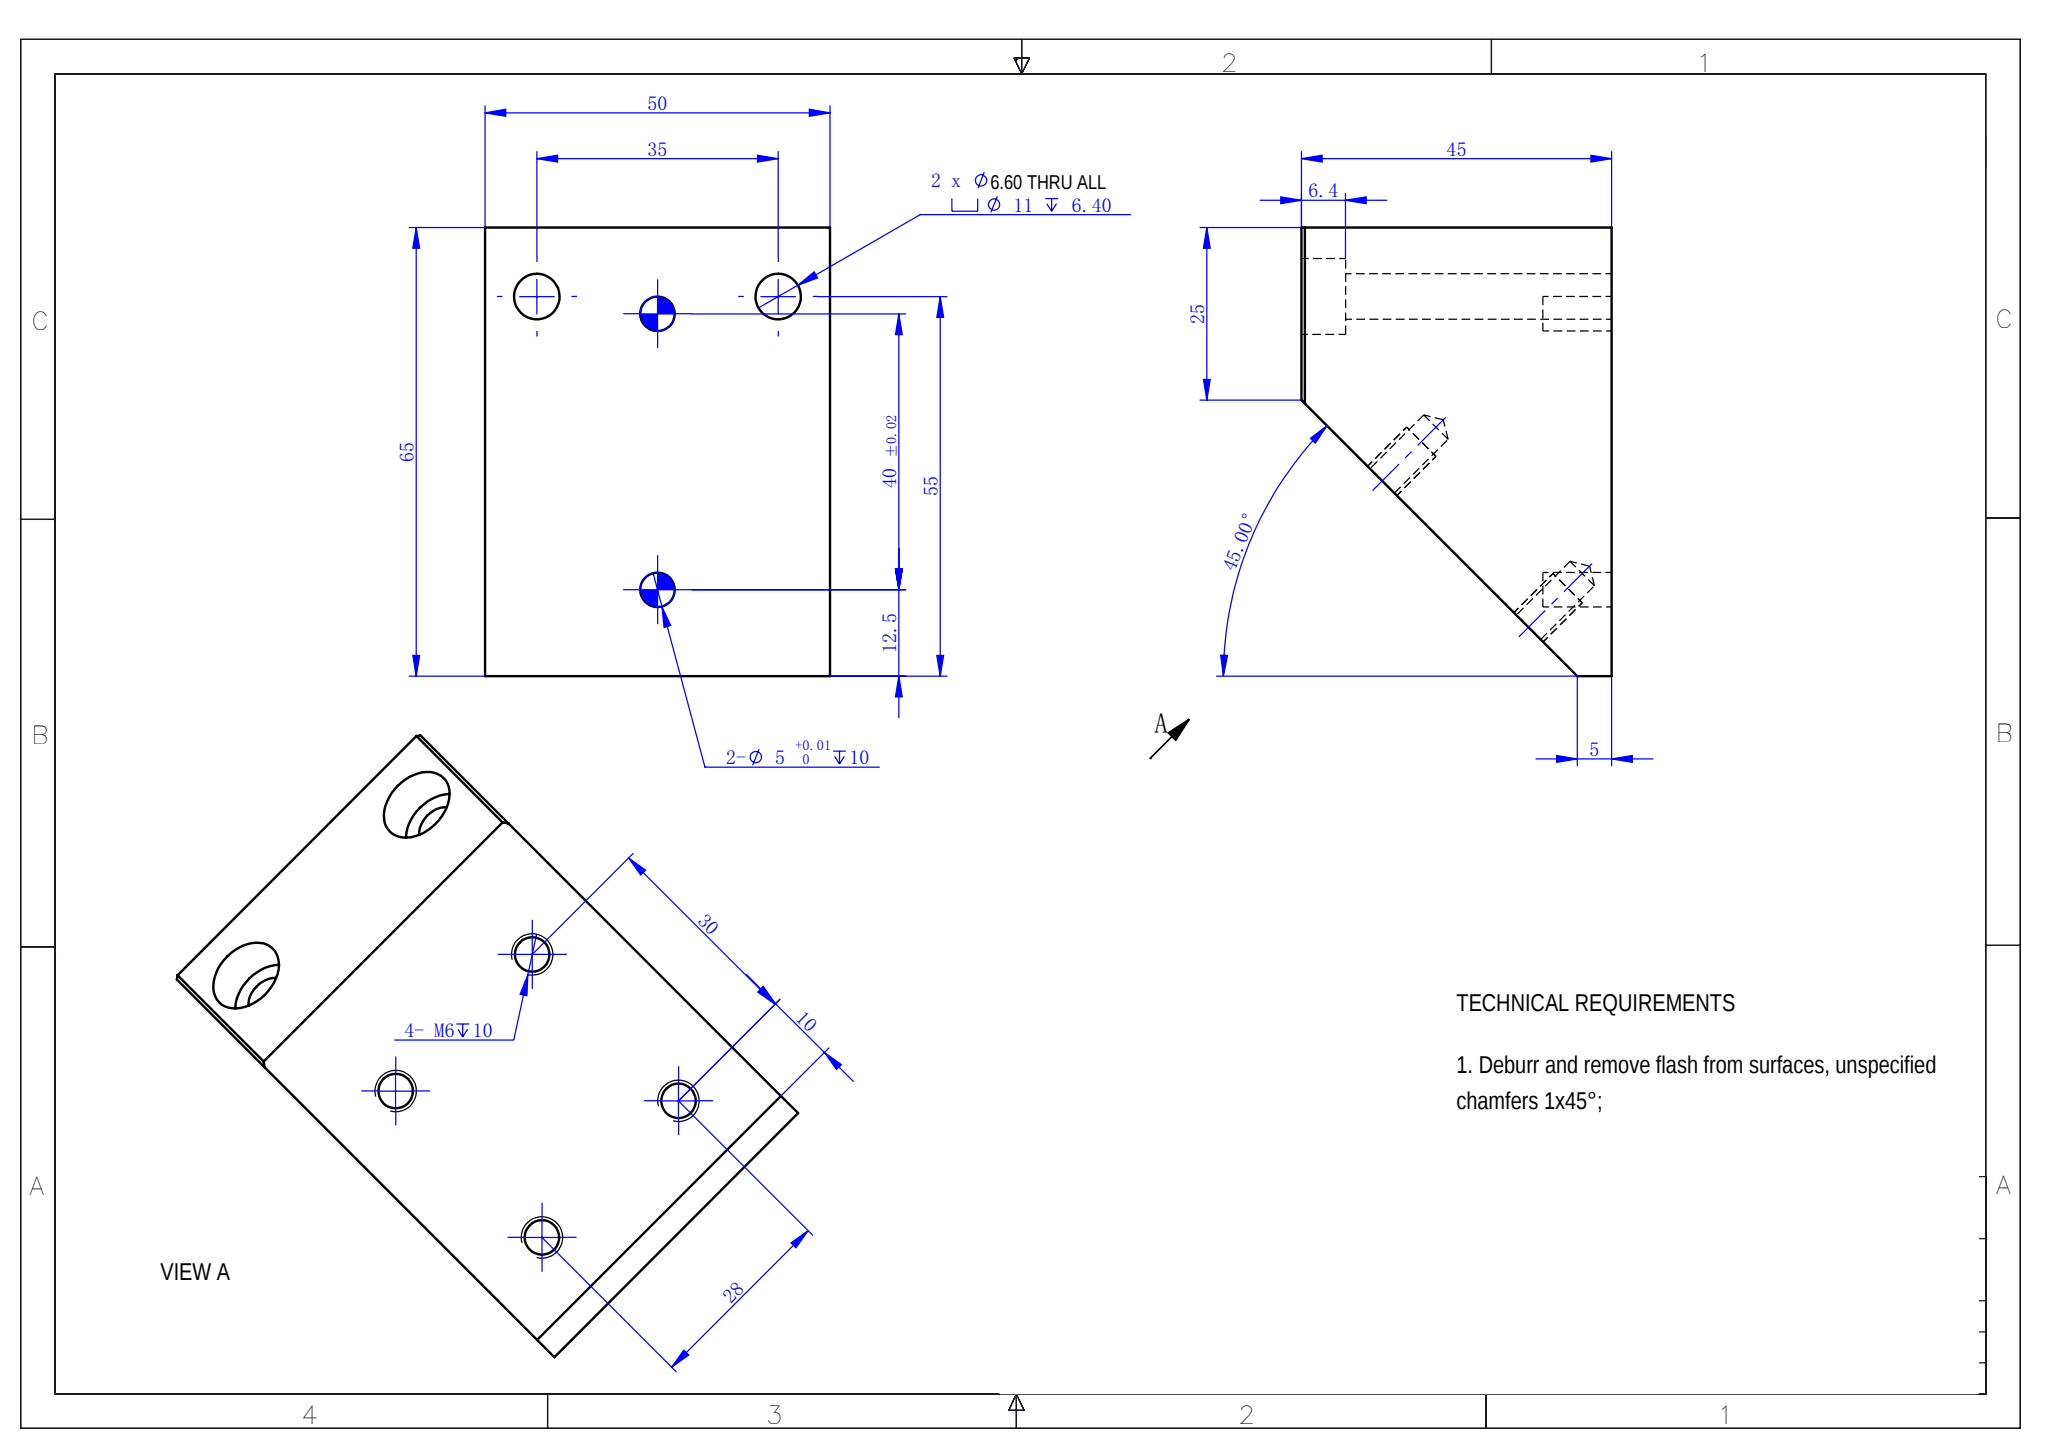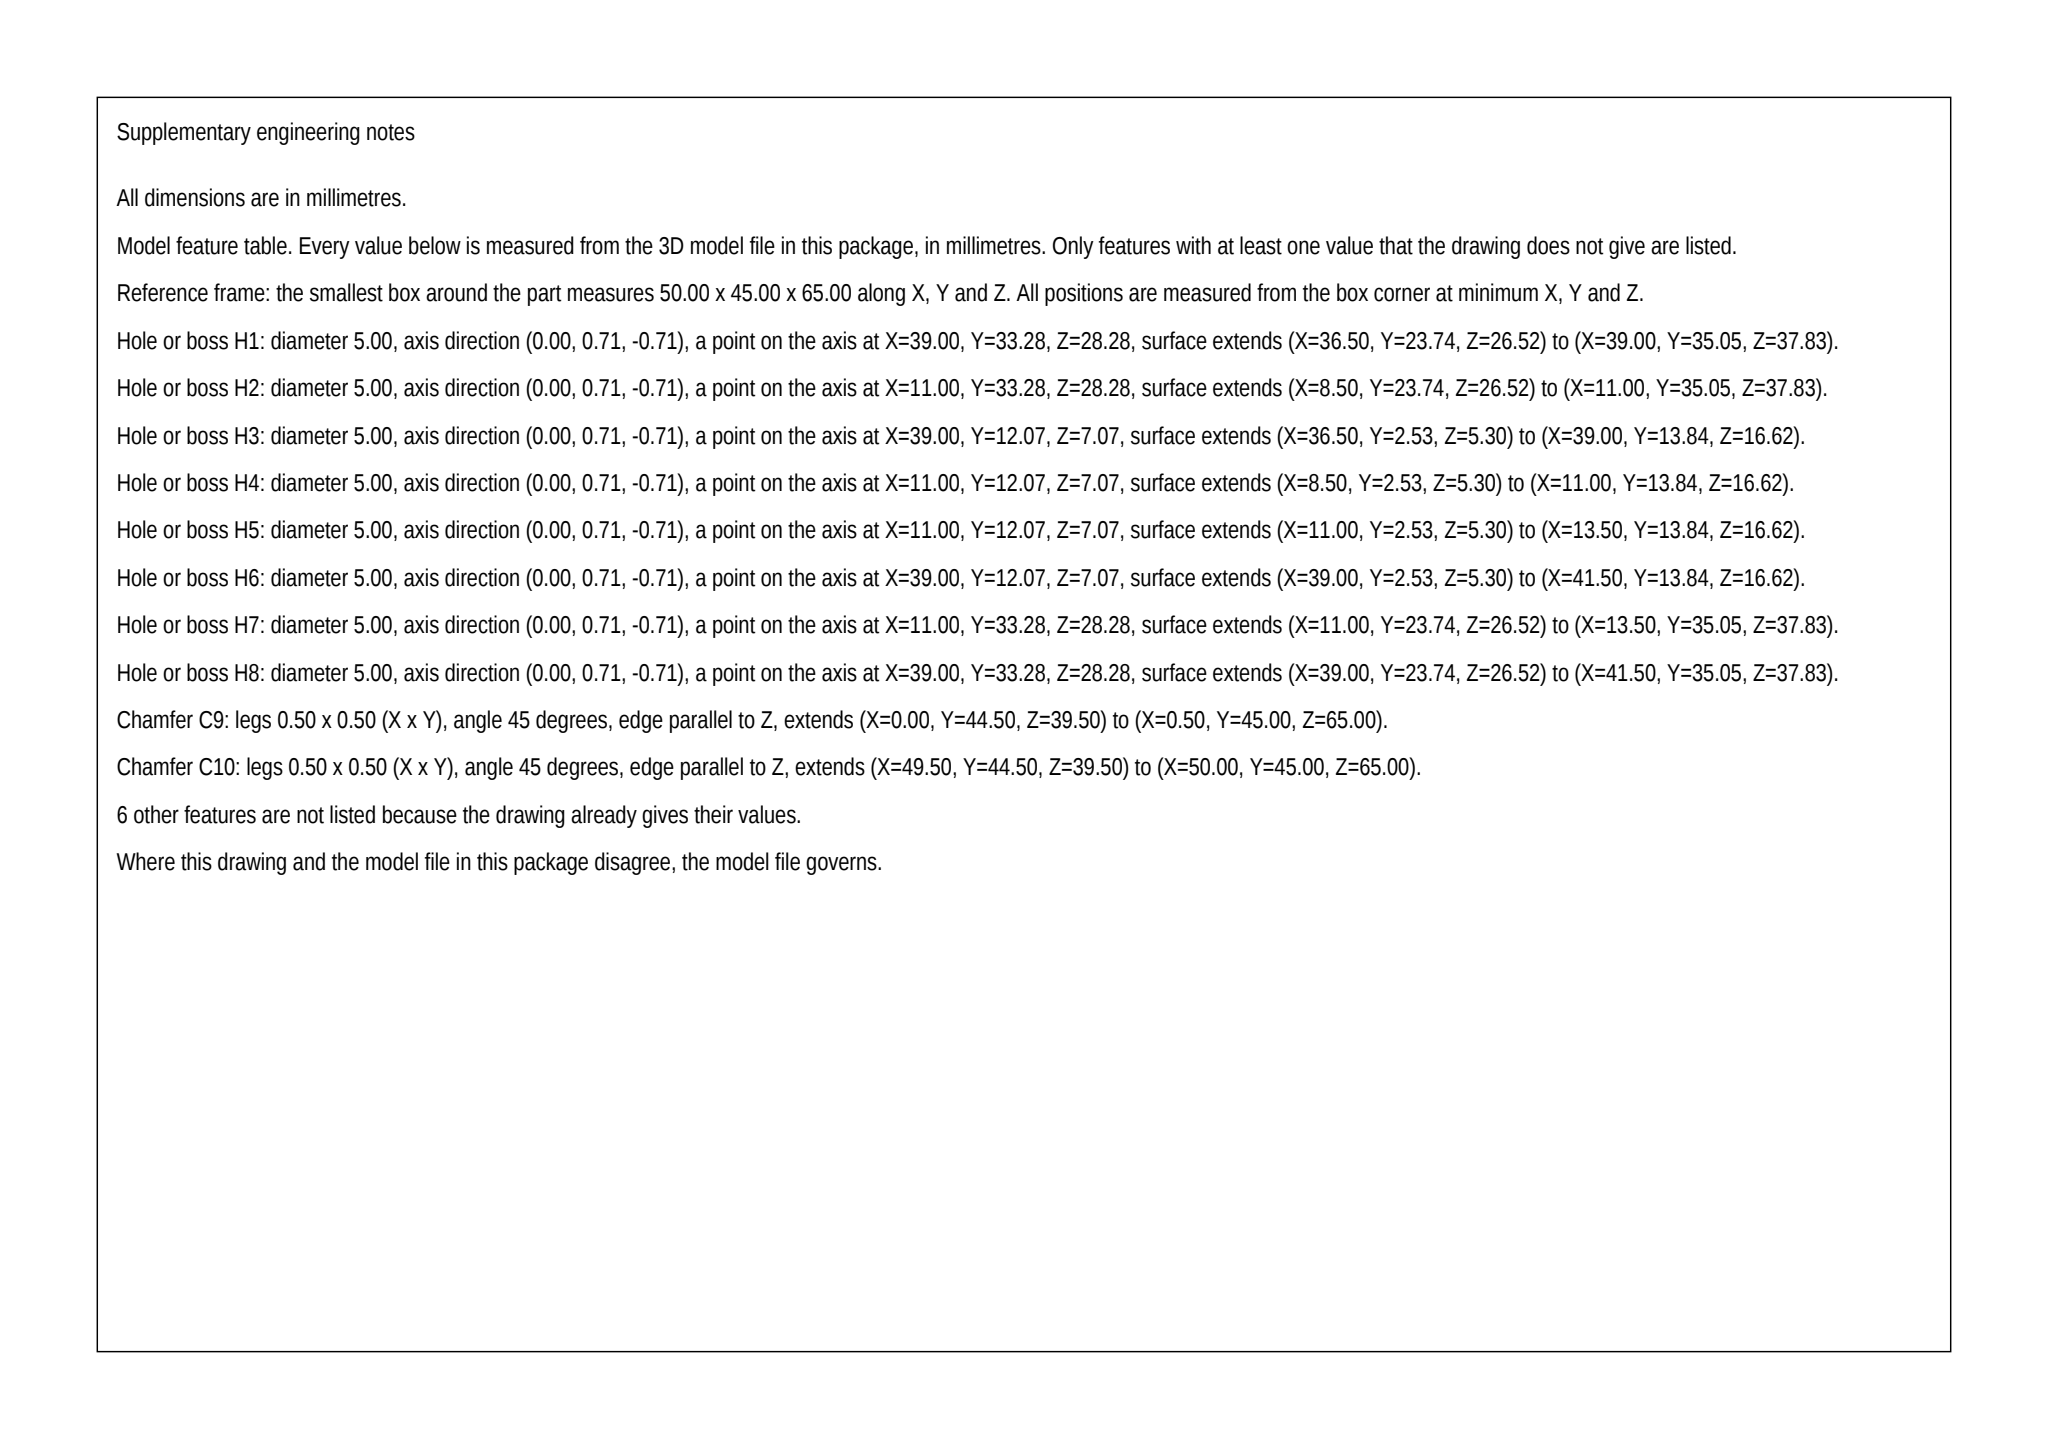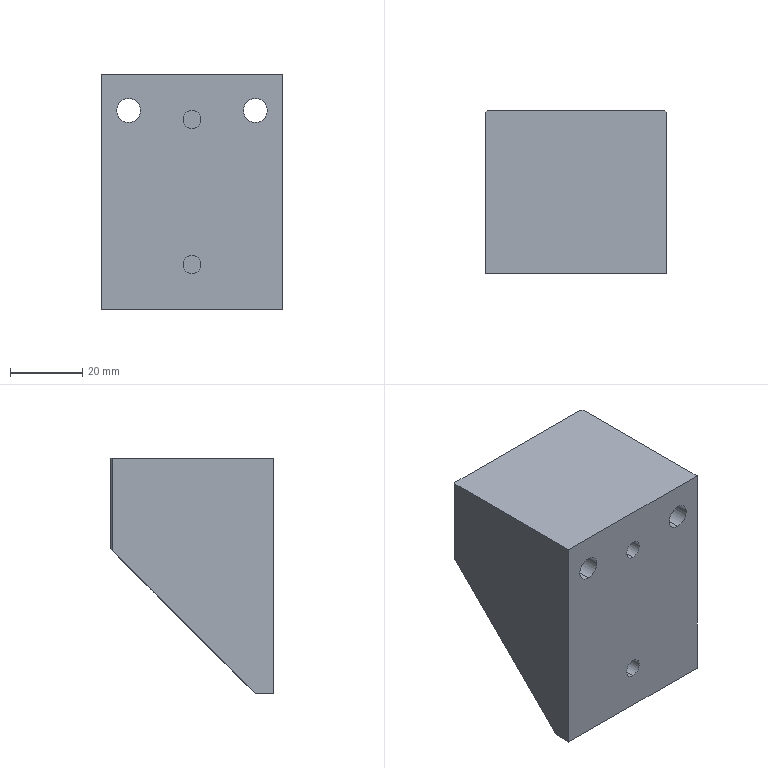Part | SolidWorks | mm | 1 solid | 41 faces | box 50 x 45 x 65 mm | volume 101090 mm3 | cylinder 20 | plane 13 | cone 8 | commonest cylinder face diameters 5 x12 11 x4 6.6 x4
build123d program:
from build123d import *

# Parameters (mm, degrees)
SKETCH1_W                                       = 50
SKETCH1_H                                       = 45
BOSS_EXTRUDE1_DEPTH                             = 65
CHAMFER1_SIZE                                   = 0.5
CUT_EXTRUDE1_DEPTH                              = 86.037
M6_TAPPED_HOLE1_D                               = 5
M6_TAPPED_HOLE1_DEPTH                           = 11
M6_TAPPED_HOLE1_TIP                             = 1.502
M6_HEX_SOCKET_HEAD_CAP_SCREW_CBORE1_D           = 6.6
M6_HEX_SOCKET_HEAD_CAP_SCREW_CBORE1_CBORE_D     = 11
M6_HEX_SOCKET_HEAD_CAP_SCREW_CBORE1_CBORE_DEPTH = 6.4
SIZE_MM_DOWEL_PIN_HOLE2_D                       = 5
SIZE_MM_DOWEL_PIN_HOLE2_DEPTH                   = 10


with BuildPart() as part:
    # Sketch1 → Boss-Extrude1 (new body)
    with BuildSketch(Plane.XY):
        Rectangle(SKETCH1_W, SKETCH1_H)
    extrude(amount=BOSS_EXTRUDE1_DEPTH)

    # Chamfer1
    chamfer1_edges = [part.edges().sort_by_distance(p)[0] for p in [
        (-25, 22.5, 32.5),
        (25, 22.5, 32.5),
    ]]
    chamfer(chamfer1_edges, length=CHAMFER1_SIZE)

    # Sketch2 → Cut-Extrude1 (cut, through all)
    with BuildSketch(Plane(origin=(25, 0, 0), x_dir=(0, 0, -1), z_dir=(1, 0, 0))):
        Polygon((0, 22.5), (-40, 22.5), (0, -17.5), align=None)
    extrude(amount=-CUT_EXTRUDE1_DEPTH, mode=Mode.SUBTRACT)

    # M6 Tapped Hole1
    with Locations(Plane(origin=(0, -8.75, 8.75), x_dir=(-1, 0, 0), z_dir=(0, 0.7071, -0.7071))):
        with Locations((-14, 27.626), (14, 27.626), (-14, -2.374), (14, -2.374)):
            Hole(M6_TAPPED_HOLE1_D / 2, depth=M6_TAPPED_HOLE1_DEPTH)
            with Locations((0, 0, -(M6_TAPPED_HOLE1_DEPTH + M6_TAPPED_HOLE1_TIP / 2))):  # 118° drill point
                Cone(0, M6_TAPPED_HOLE1_D / 2, M6_TAPPED_HOLE1_TIP, mode=Mode.SUBTRACT)

    # M6 Hex Socket Head Cap Screw CBORE1 (through all)
    with Locations(Plane(origin=(0, 22.5, 0), x_dir=(1, 0, 0), z_dir=(0, 1, 0))):
        with Locations((17.5, -55), (-17.5, -55)):
            CounterBoreHole(M6_HEX_SOCKET_HEAD_CAP_SCREW_CBORE1_D / 2, M6_HEX_SOCKET_HEAD_CAP_SCREW_CBORE1_CBORE_D / 2, M6_HEX_SOCKET_HEAD_CAP_SCREW_CBORE1_CBORE_DEPTH)

    # Size mm Dowel Pin Hole2
    with Locations(Plane(origin=(0, -22.5, 0), x_dir=(-1, 0, 0), z_dir=(0, -1, 0))):
        with Locations((0, -12.5), (0, -52.5)):
            Hole(SIZE_MM_DOWEL_PIN_HOLE2_D / 2, depth=SIZE_MM_DOWEL_PIN_HOLE2_DEPTH)


solid = part.part